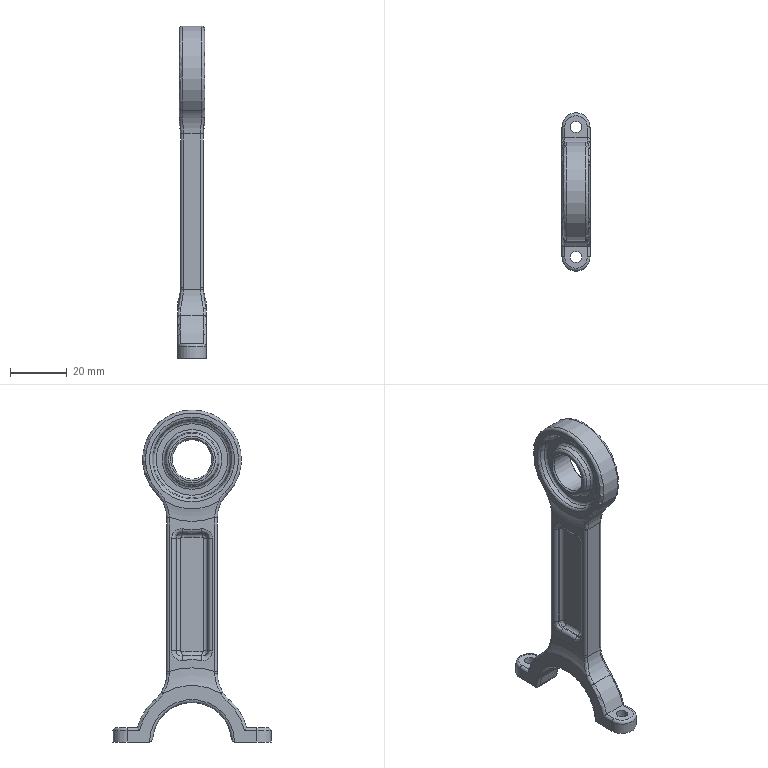Component | NX | CON_ROD_4 | 1 solid | 141 faces | volume 16005 mm3 | torus 42 | spline 36 | cylinder 31 | plane 22 | cone 10 | commonest cylinder face diameters 2 x8 3 x8 24 x4 40 x2 10 x2 4 x2 2.4 x2 28 x1